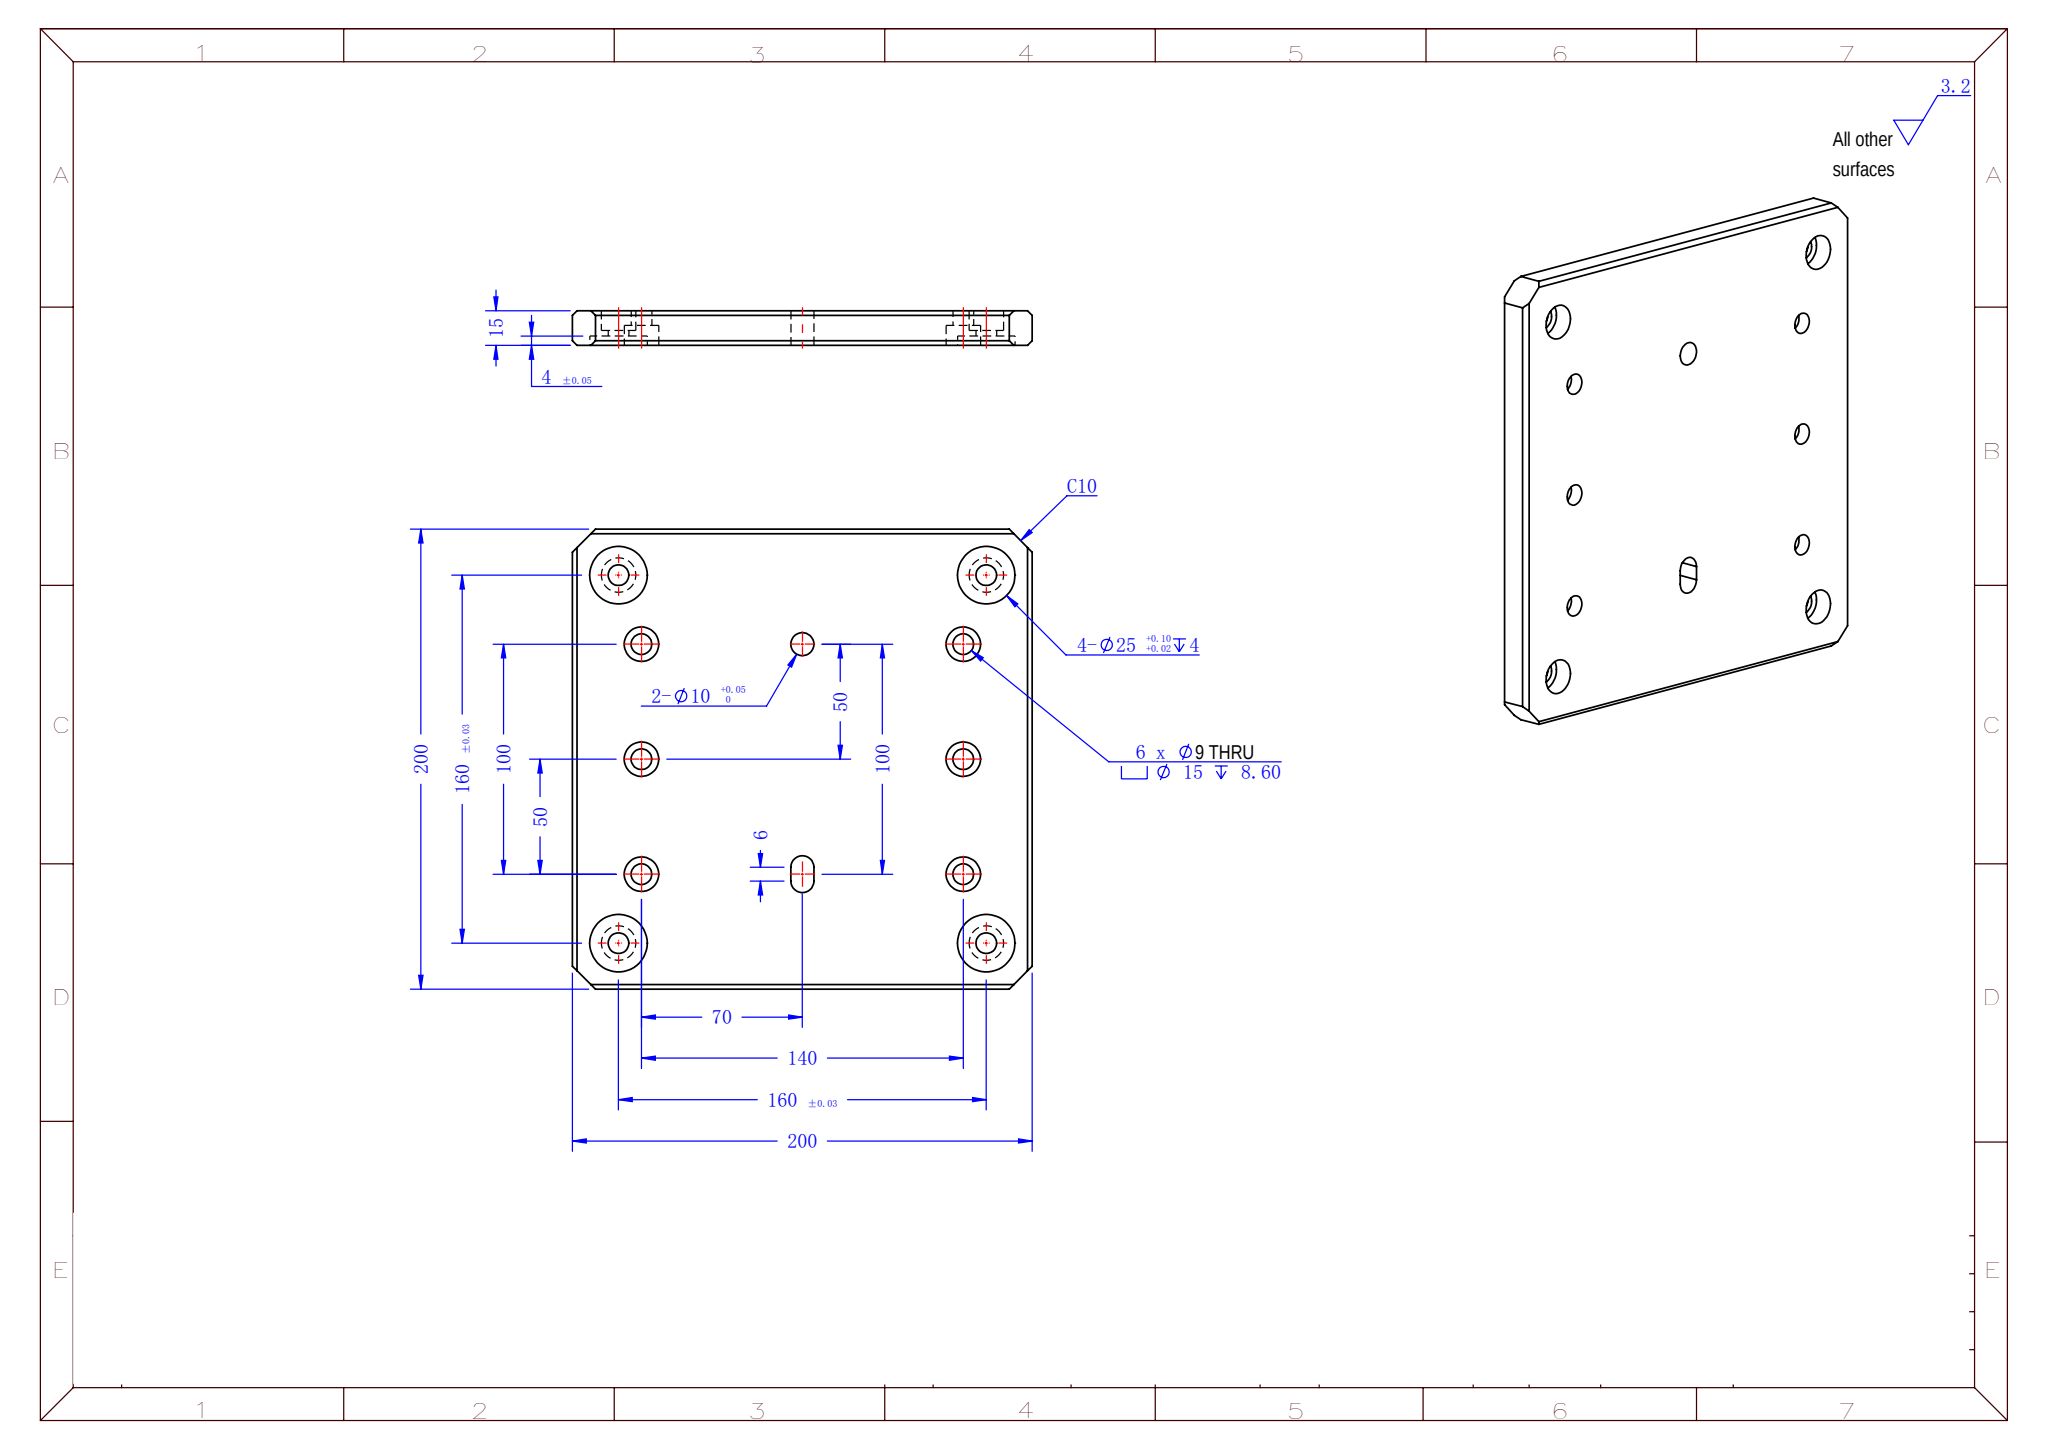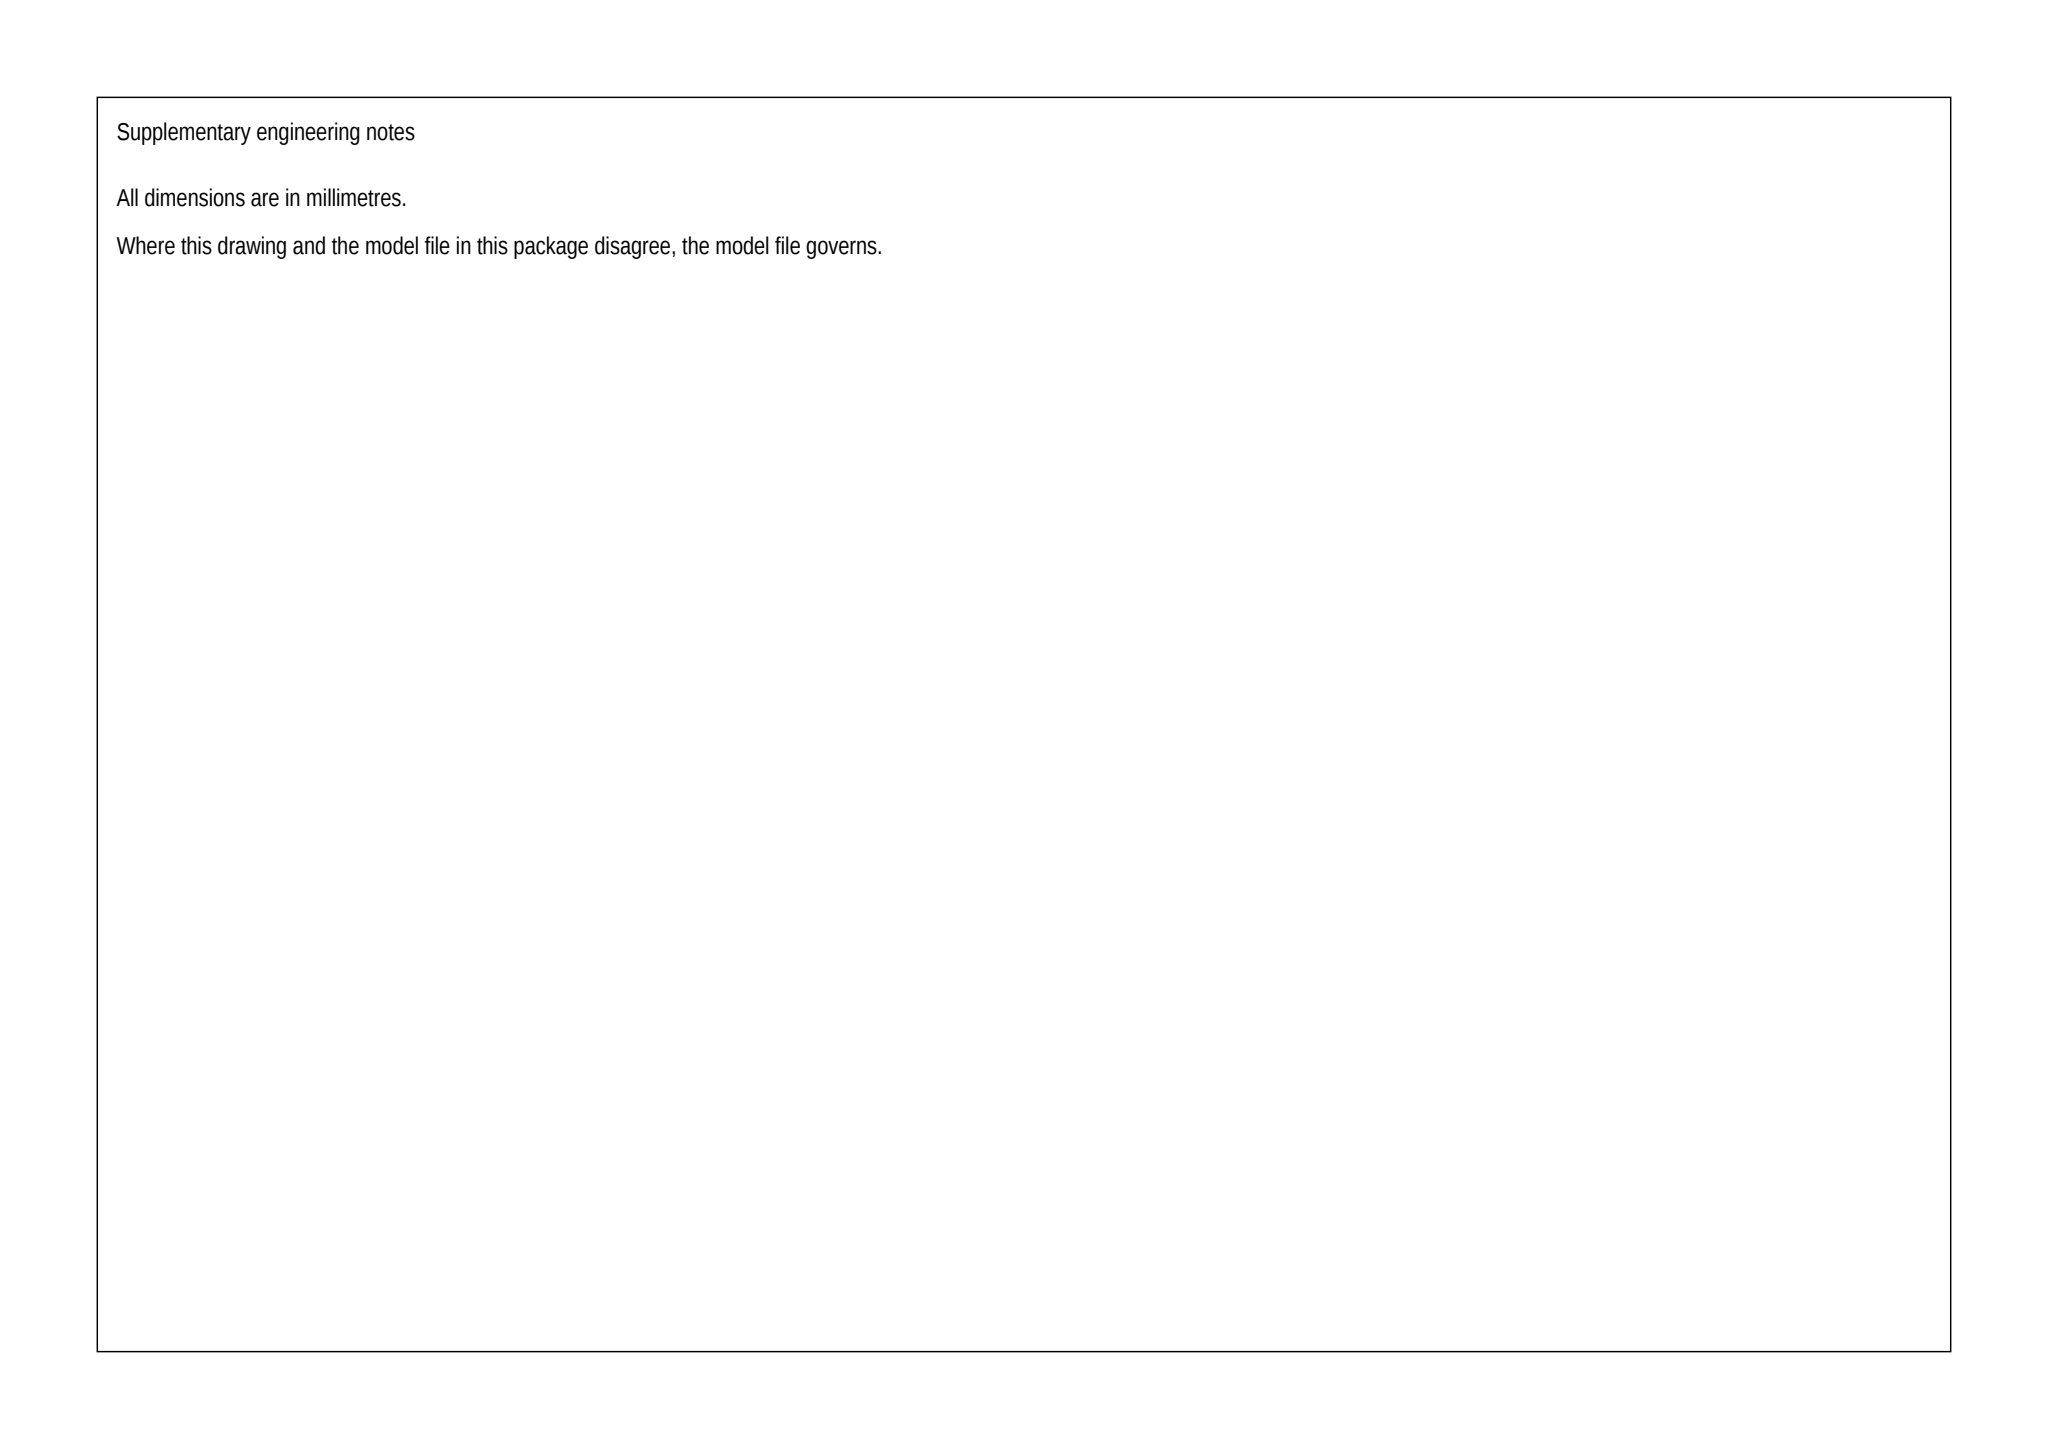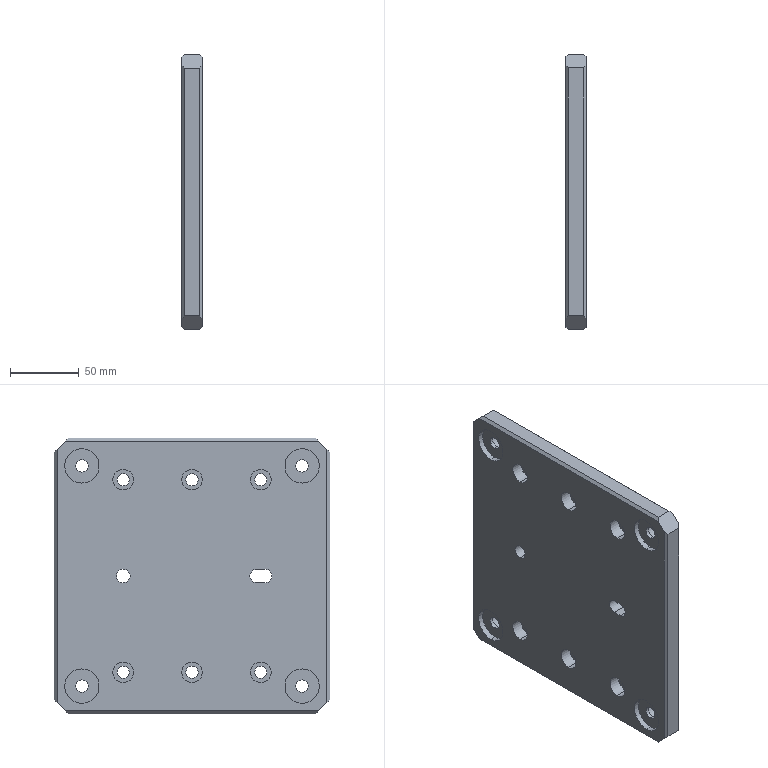Part | SolidWorks | mm | 1 solid | 86 faces | box 15 x 200 x 200 mm | volume 564737 mm3 | cylinder 52 | plane 34 | commonest cylinder face diameters 15 x20 9 x20 25 x8 10 x4
Drawing notes:
4 CORNER HOLES: Ø9 THRU, C'BORE Ø15 DP 8.60 OPP Ø25 DP 4 | from the solid: Ø9 L2.4 + Ø15 L8.6 + Ø25 L4 = 15 thk at (20,20),(20,180),(180,20),(180,180)
Ø25 DP 4 FROM FRONT FACE; ALL Ø15 DP 8.60 FROM OPP FACE | from the solid: Ø25 bores start x=0 face (planes x=4); Ø15 bores start x=15 face (planes x=8.6/6.4)
build123d program:
from build123d import *

# Parameters (mm, degrees)
SKETCH1_W                                       = 200
SKETCH1_H                                       = 200
BOSS_EXTRUDE1_DEPTH                             = 15
CHAMFER1_SIZE                                   = 10
M8_HEX_SOCKET_HEAD_CAP_SCREW_CBORE1_D           = 9
M8_HEX_SOCKET_HEAD_CAP_SCREW_CBORE1_CBORE_D     = 15
M8_HEX_SOCKET_HEAD_CAP_SCREW_CBORE1_CBORE_DEPTH = 8.6
SKETCH4_R                                       = 12.5
CUT_EXTRUDE1_DEPTH                              = 4
M8_HEX_SOCKET_HEAD_CAP_SCREW_CBORE2_D           = 9
M8_HEX_SOCKET_HEAD_CAP_SCREW_CBORE2_CBORE_D     = 15
M8_HEX_SOCKET_HEAD_CAP_SCREW_CBORE2_CBORE_DEPTH = 8.6
CUT_EXTRUDE2_REACH                              = 144.215
SKETCH7_R                                       = 5
CHAMFER2_SIZE                                   = 2


with BuildPart() as part:
    # Sketch1 → Boss-Extrude1 (new body)
    with BuildSketch(Plane(origin=(0, 0, 0), x_dir=(0, 0, -1), z_dir=(1, 0, 0))):
        Rectangle(SKETCH1_W, SKETCH1_H)
    extrude(amount=BOSS_EXTRUDE1_DEPTH)

    # Chamfer1
    chamfer1_edges = [part.edges().sort_by_distance(p)[0] for p in [
        (7.5, -100, -100),
        (7.5, -100, 100),
        (7.5, 100, 100),
        (7.5, 100, -100),
    ]]
    chamfer(chamfer1_edges, length=CHAMFER1_SIZE)

    # M8 Hex Socket Head Cap Screw CBORE1 (through all)
    with Locations(Plane(origin=(15, 0, 0), x_dir=(0, 0, -1), z_dir=(1, 0, 0))):
        with Locations((-80, 80), (80, 80), (80, -80), (-80, -80)):
            CounterBoreHole(M8_HEX_SOCKET_HEAD_CAP_SCREW_CBORE1_D / 2, M8_HEX_SOCKET_HEAD_CAP_SCREW_CBORE1_CBORE_D / 2, M8_HEX_SOCKET_HEAD_CAP_SCREW_CBORE1_CBORE_DEPTH)

    # Sketch4 → Cut-Extrude1 (cut)
    with BuildSketch(Plane.ZY):
        with Locations((-80, 80)):
            Circle(SKETCH4_R)
        with Locations((80, 80)):
            Circle(SKETCH4_R)
        with Locations((80, -80)):
            Circle(SKETCH4_R)
        with Locations((-80, -80)):
            Circle(SKETCH4_R)
    extrude(amount=-CUT_EXTRUDE1_DEPTH, mode=Mode.SUBTRACT)

    # M8 Hex Socket Head Cap Screw CBORE2 (through all)
    with Locations(Plane.ZY):
        with Locations((-70, 50), (70, 50), (-70, -50), (70, -50), (70, 0), (-70, 0)):
            CounterBoreHole(M8_HEX_SOCKET_HEAD_CAP_SCREW_CBORE2_D / 2, M8_HEX_SOCKET_HEAD_CAP_SCREW_CBORE2_CBORE_D / 2, M8_HEX_SOCKET_HEAD_CAP_SCREW_CBORE2_CBORE_DEPTH)

    # Sketch7 → Cut-Extrude2 (cut, up to next)
    with BuildSketch(Plane.ZY, mode=Mode.PRIVATE) as cut_extrude2_sk1:
        with Locations((0, 50)):
            Circle(SKETCH7_R)
    cut_extrude2_tool1 = extrude(cut_extrude2_sk1.sketch, amount=-CUT_EXTRUDE2_REACH, mode=Mode.PRIVATE) & part.part
    # Sketch7 → Cut-Extrude2 (cut, up to next)
    with BuildSketch(Plane.ZY, mode=Mode.PRIVATE) as cut_extrude2_sk2:
        with BuildLine():
            Line((-5, -53), (-5, -47))
            ThreePointArc((-5, -47), (0, -42), (5, -47))
            Line((5, -47), (5, -53))
            ThreePointArc((5, -53), (0, -58), (-5, -53))
        make_face()
    cut_extrude2_tool2 = extrude(cut_extrude2_sk2.sketch, amount=-CUT_EXTRUDE2_REACH, mode=Mode.PRIVATE) & part.part
    add(cut_extrude2_tool1.solids().sort_by_distance((0, 50, 0))[0], mode=Mode.SUBTRACT)
    add(cut_extrude2_tool2.solids().sort_by_distance((0, -50, 0))[0], mode=Mode.SUBTRACT)

    # Chamfer2
    chamfer2_edges = [part.edges().sort_by_distance(p)[0] for p in [
        (0, 0, 100),
        (15, 0, 100),
        (0, 0, -100),
        (0, -100, 0),
        (0, 100, 0),
        (15, 100, 0),
        (15, 0, -100),
        (15, -100, 0),
    ]]
    chamfer(chamfer2_edges, length=CHAMFER2_SIZE)


solid = part.part